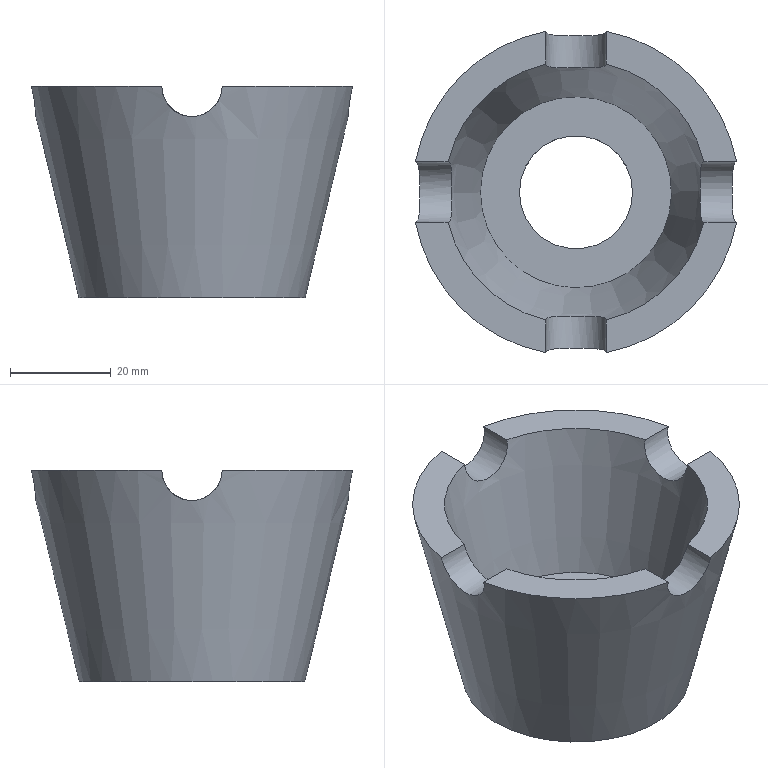Component | NX | CAP | 1 solid | 13 faces | volume 46250 mm3 | plane 6 | cylinder 5 | cone 2 | commonest cylinder face diameters 12 x4 22.5 x1